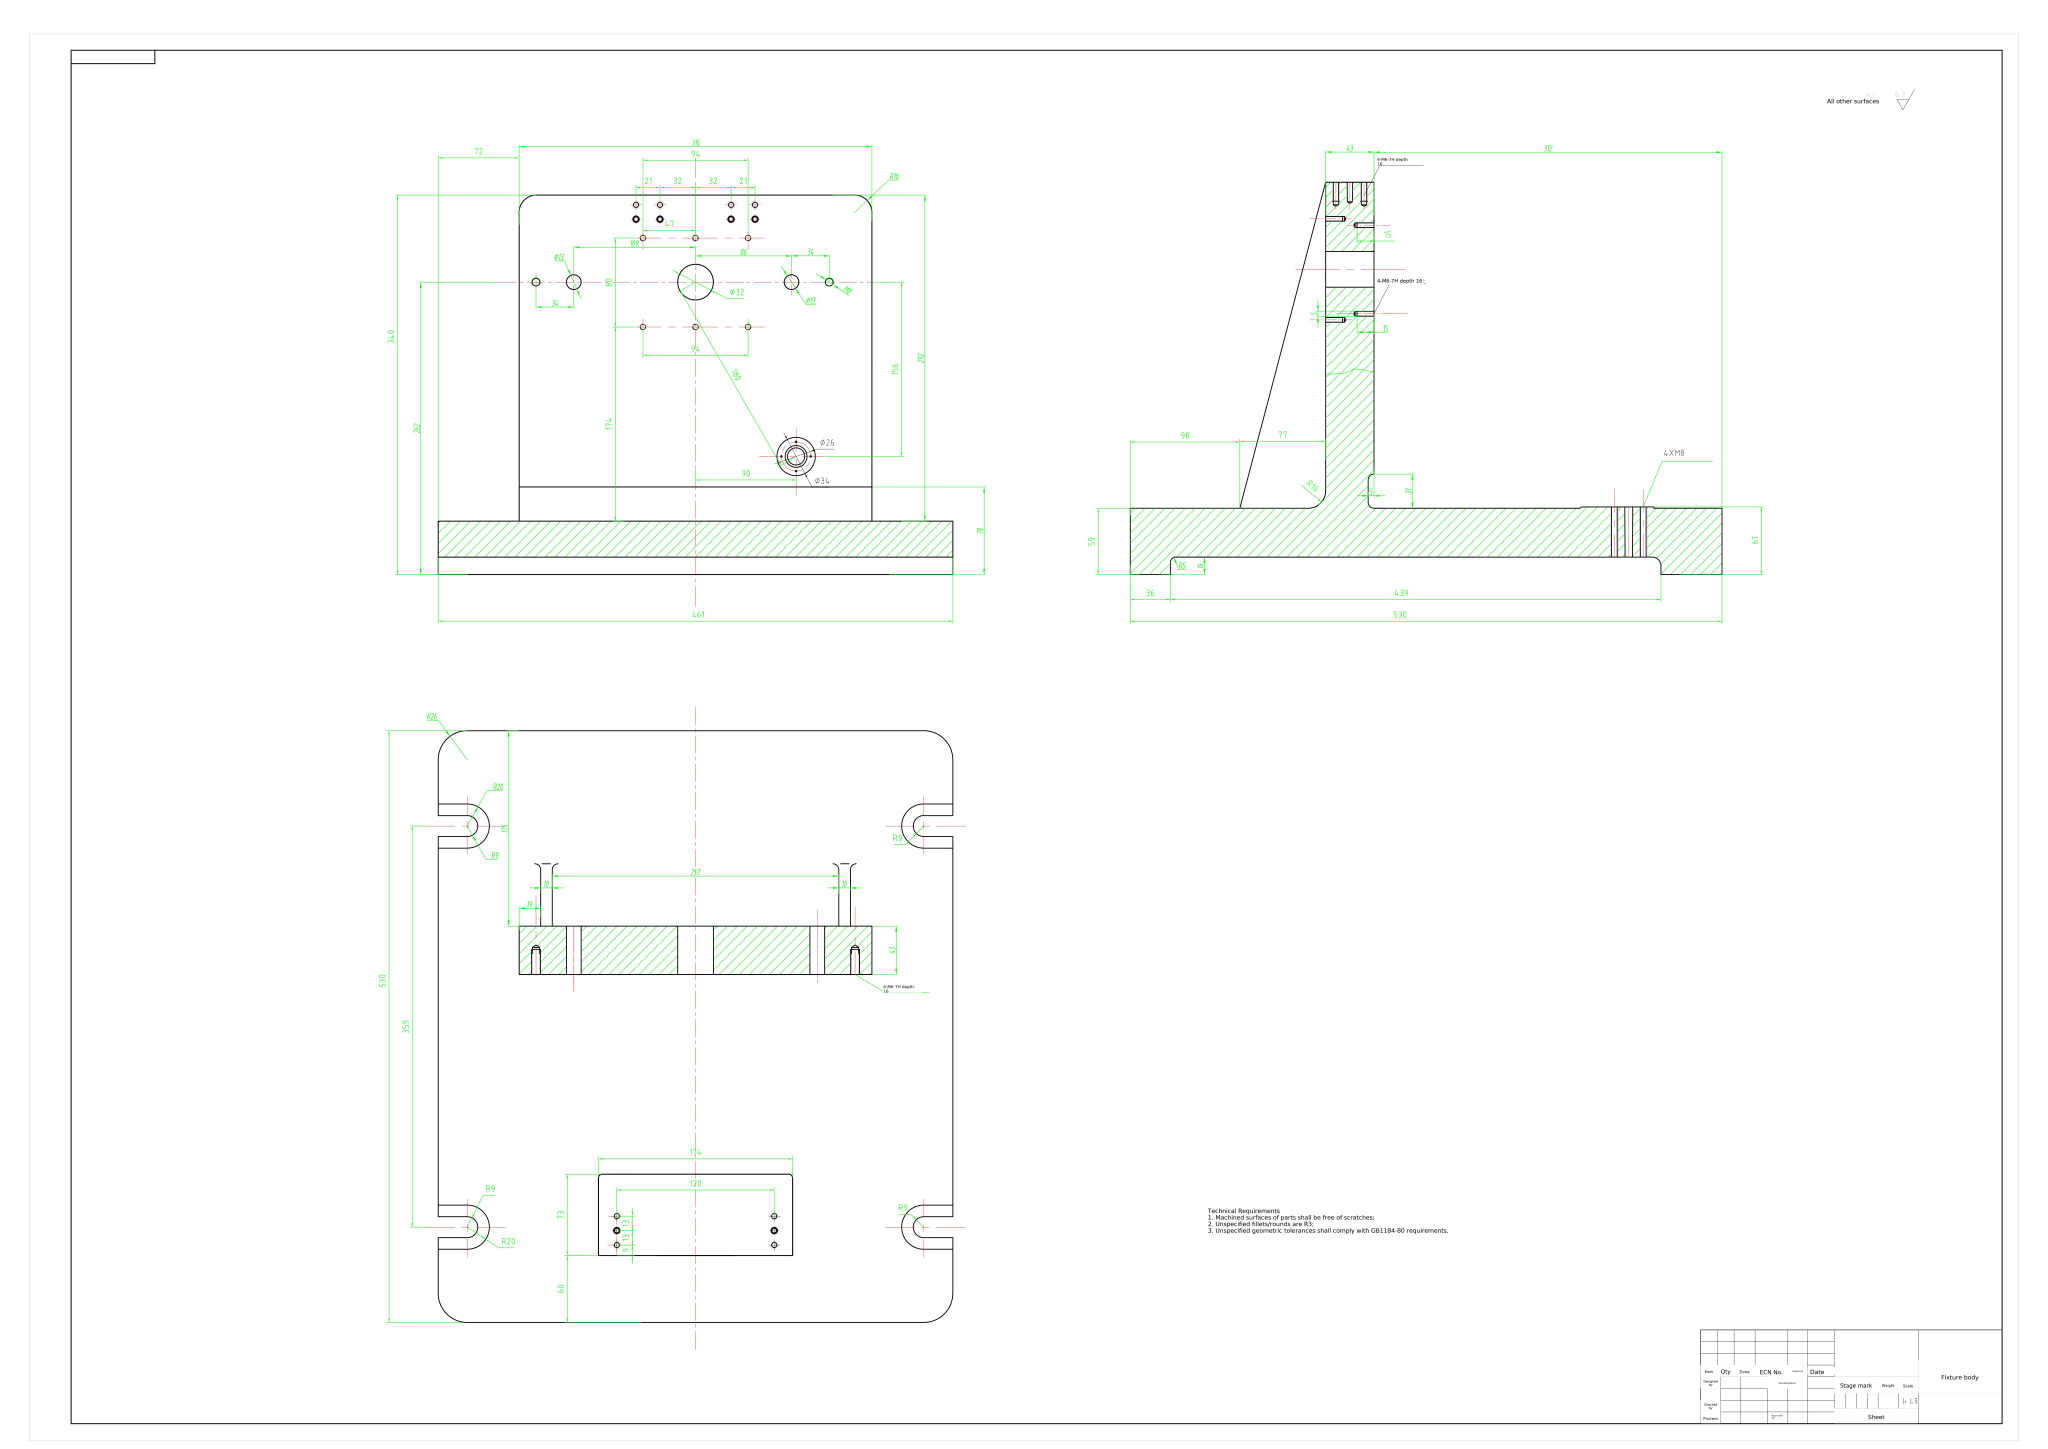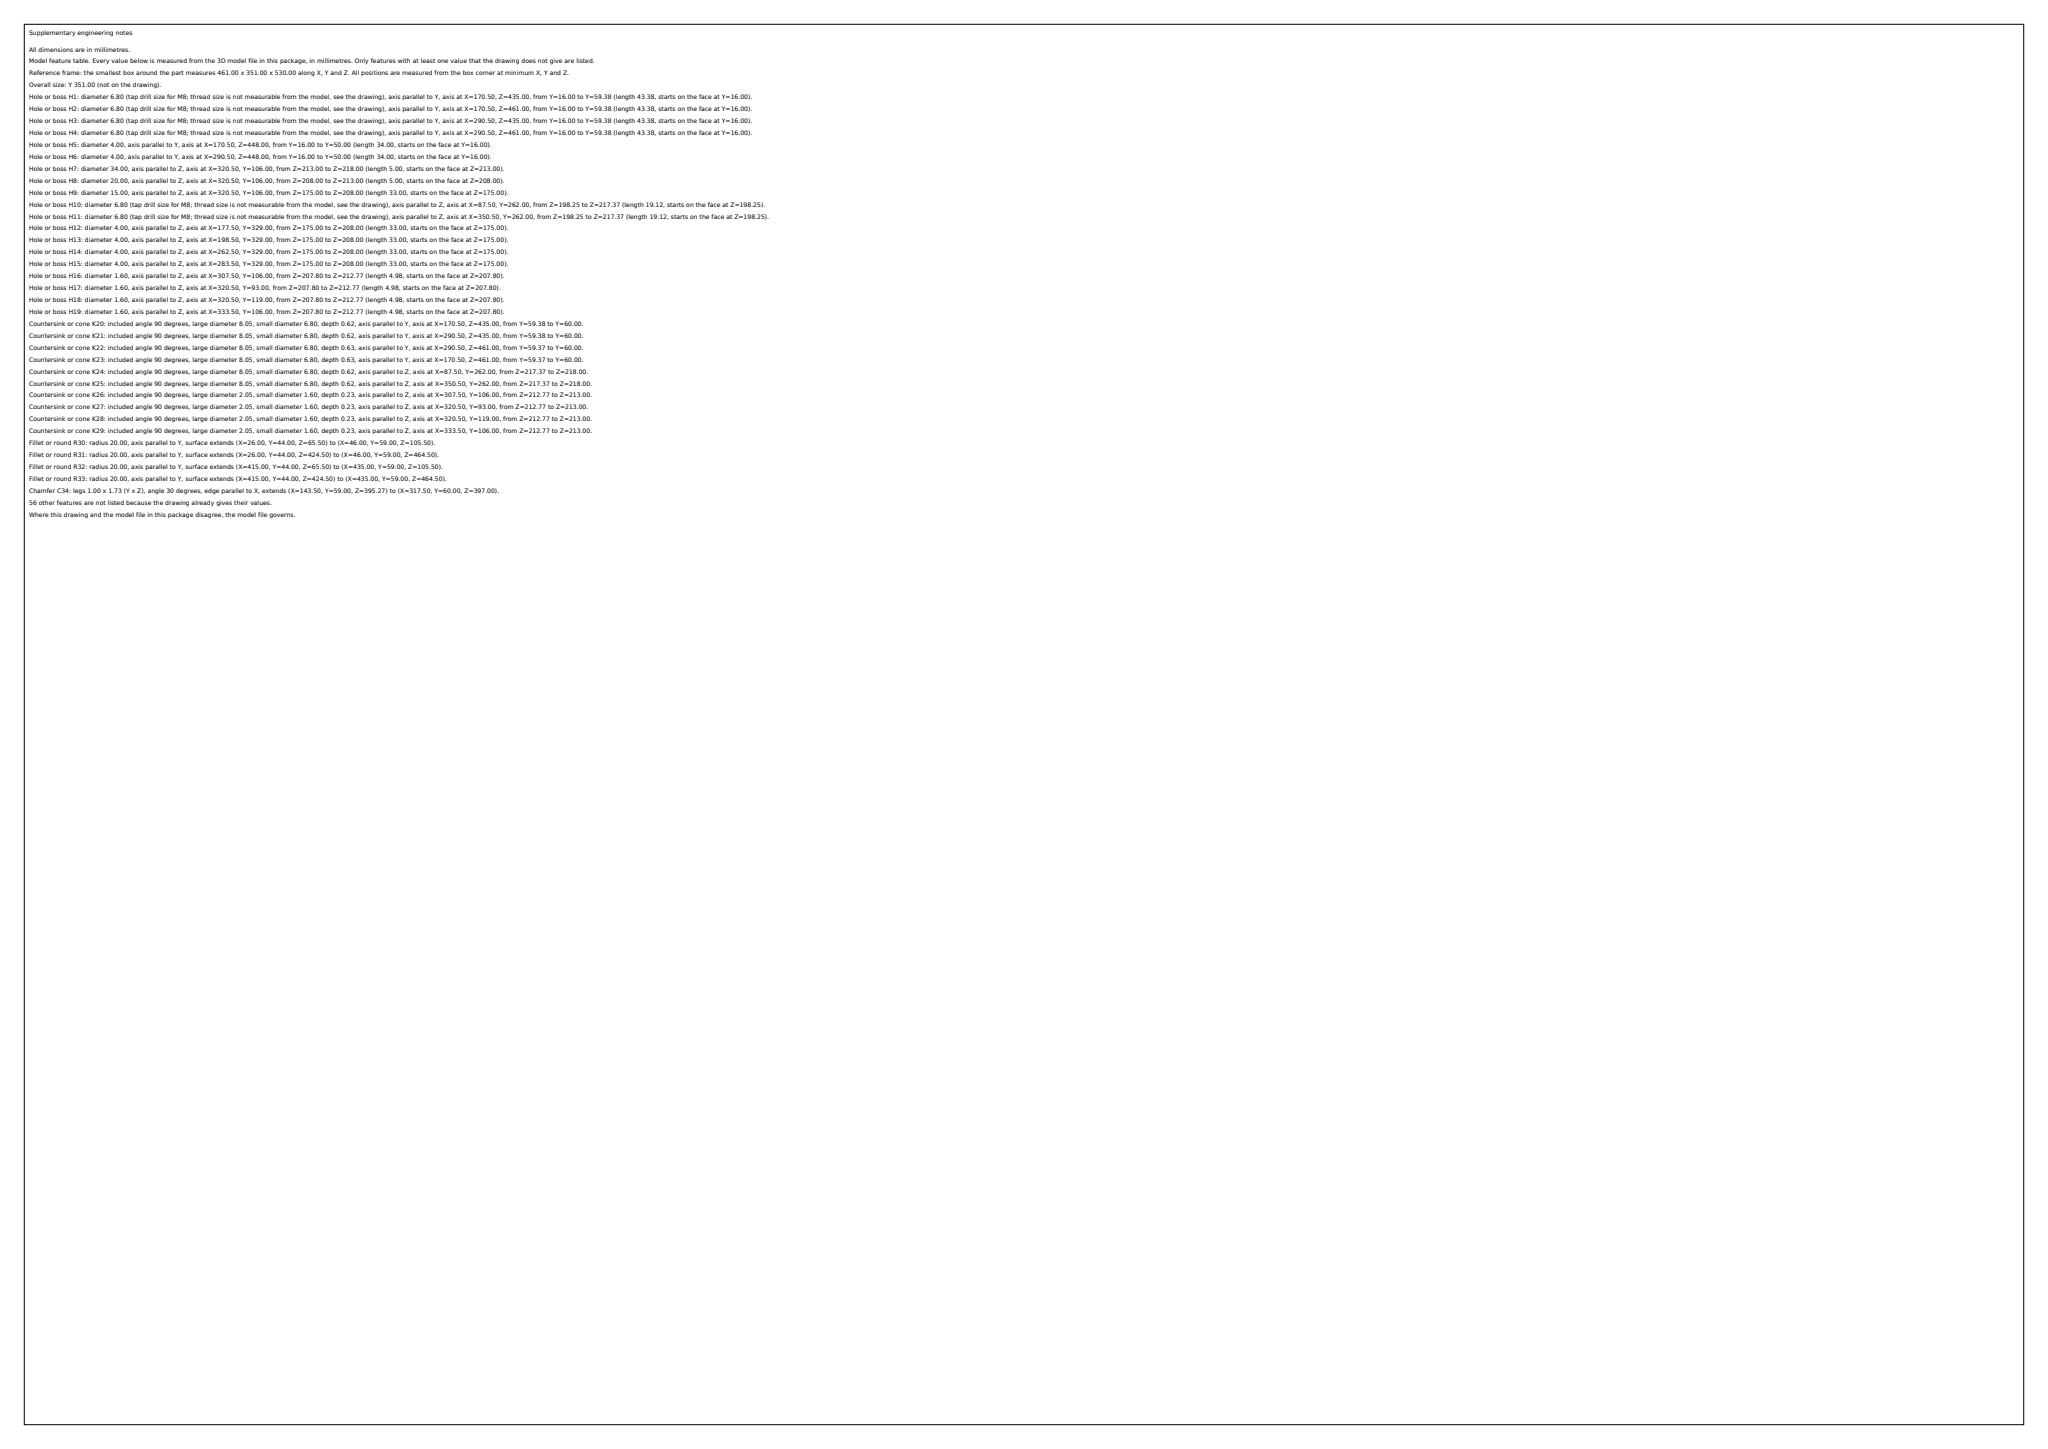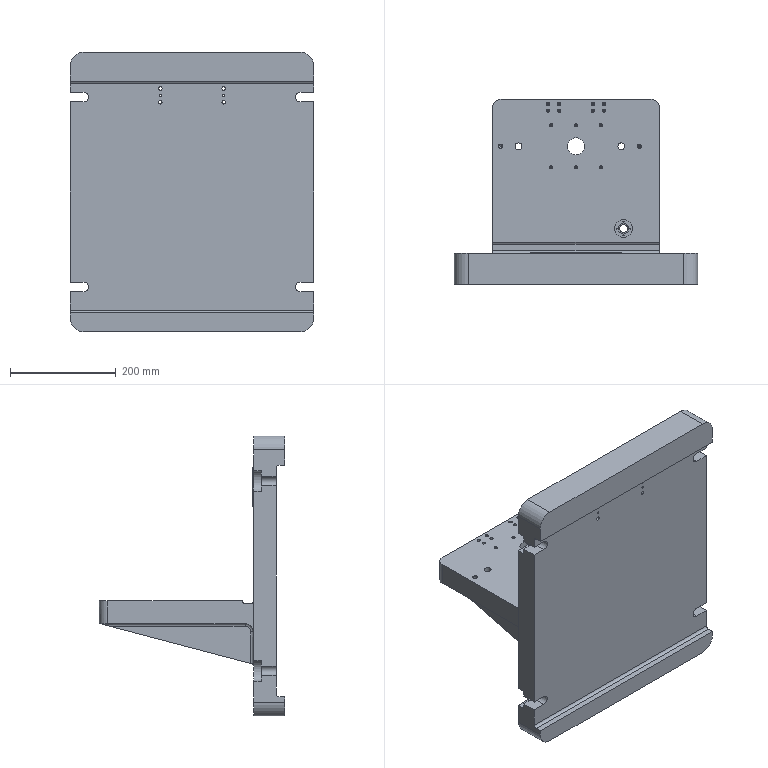Part | SolidWorks | mm | 1 solid | 242 faces | box 461 x 351 x 530 mm | volume 15102961 mm3 | cylinder 105 | cone 72 | plane 61 | torus 4 | commonest cylinder face diameters 5 x20 6.8 x12 6 x12 4 x12 10 x12 1.6 x8 32 x7 13 x4